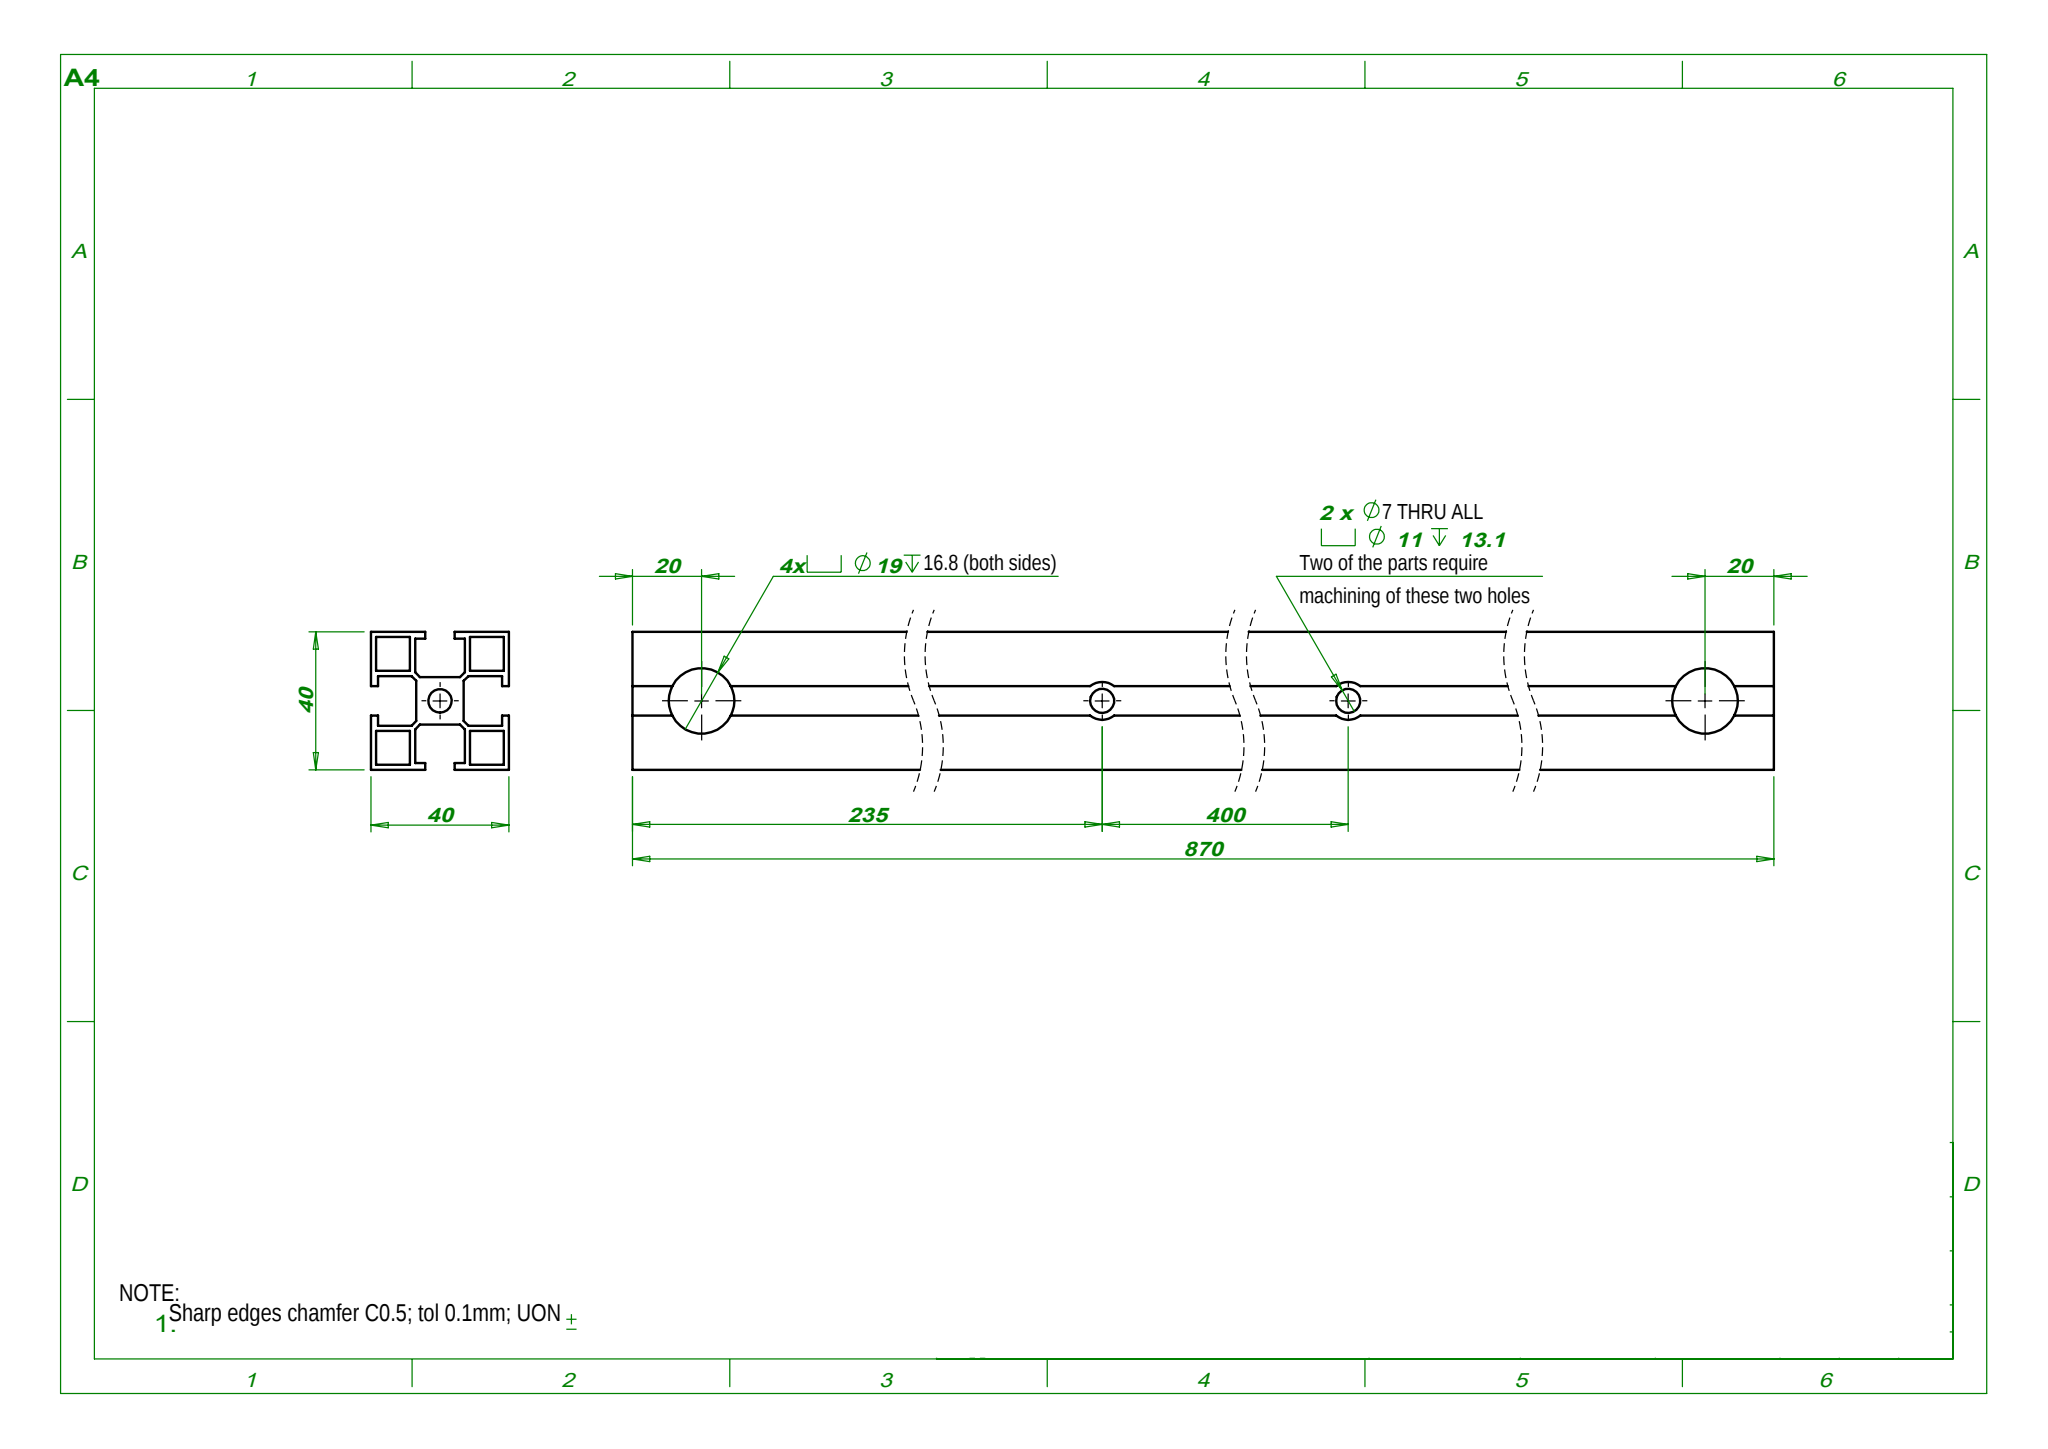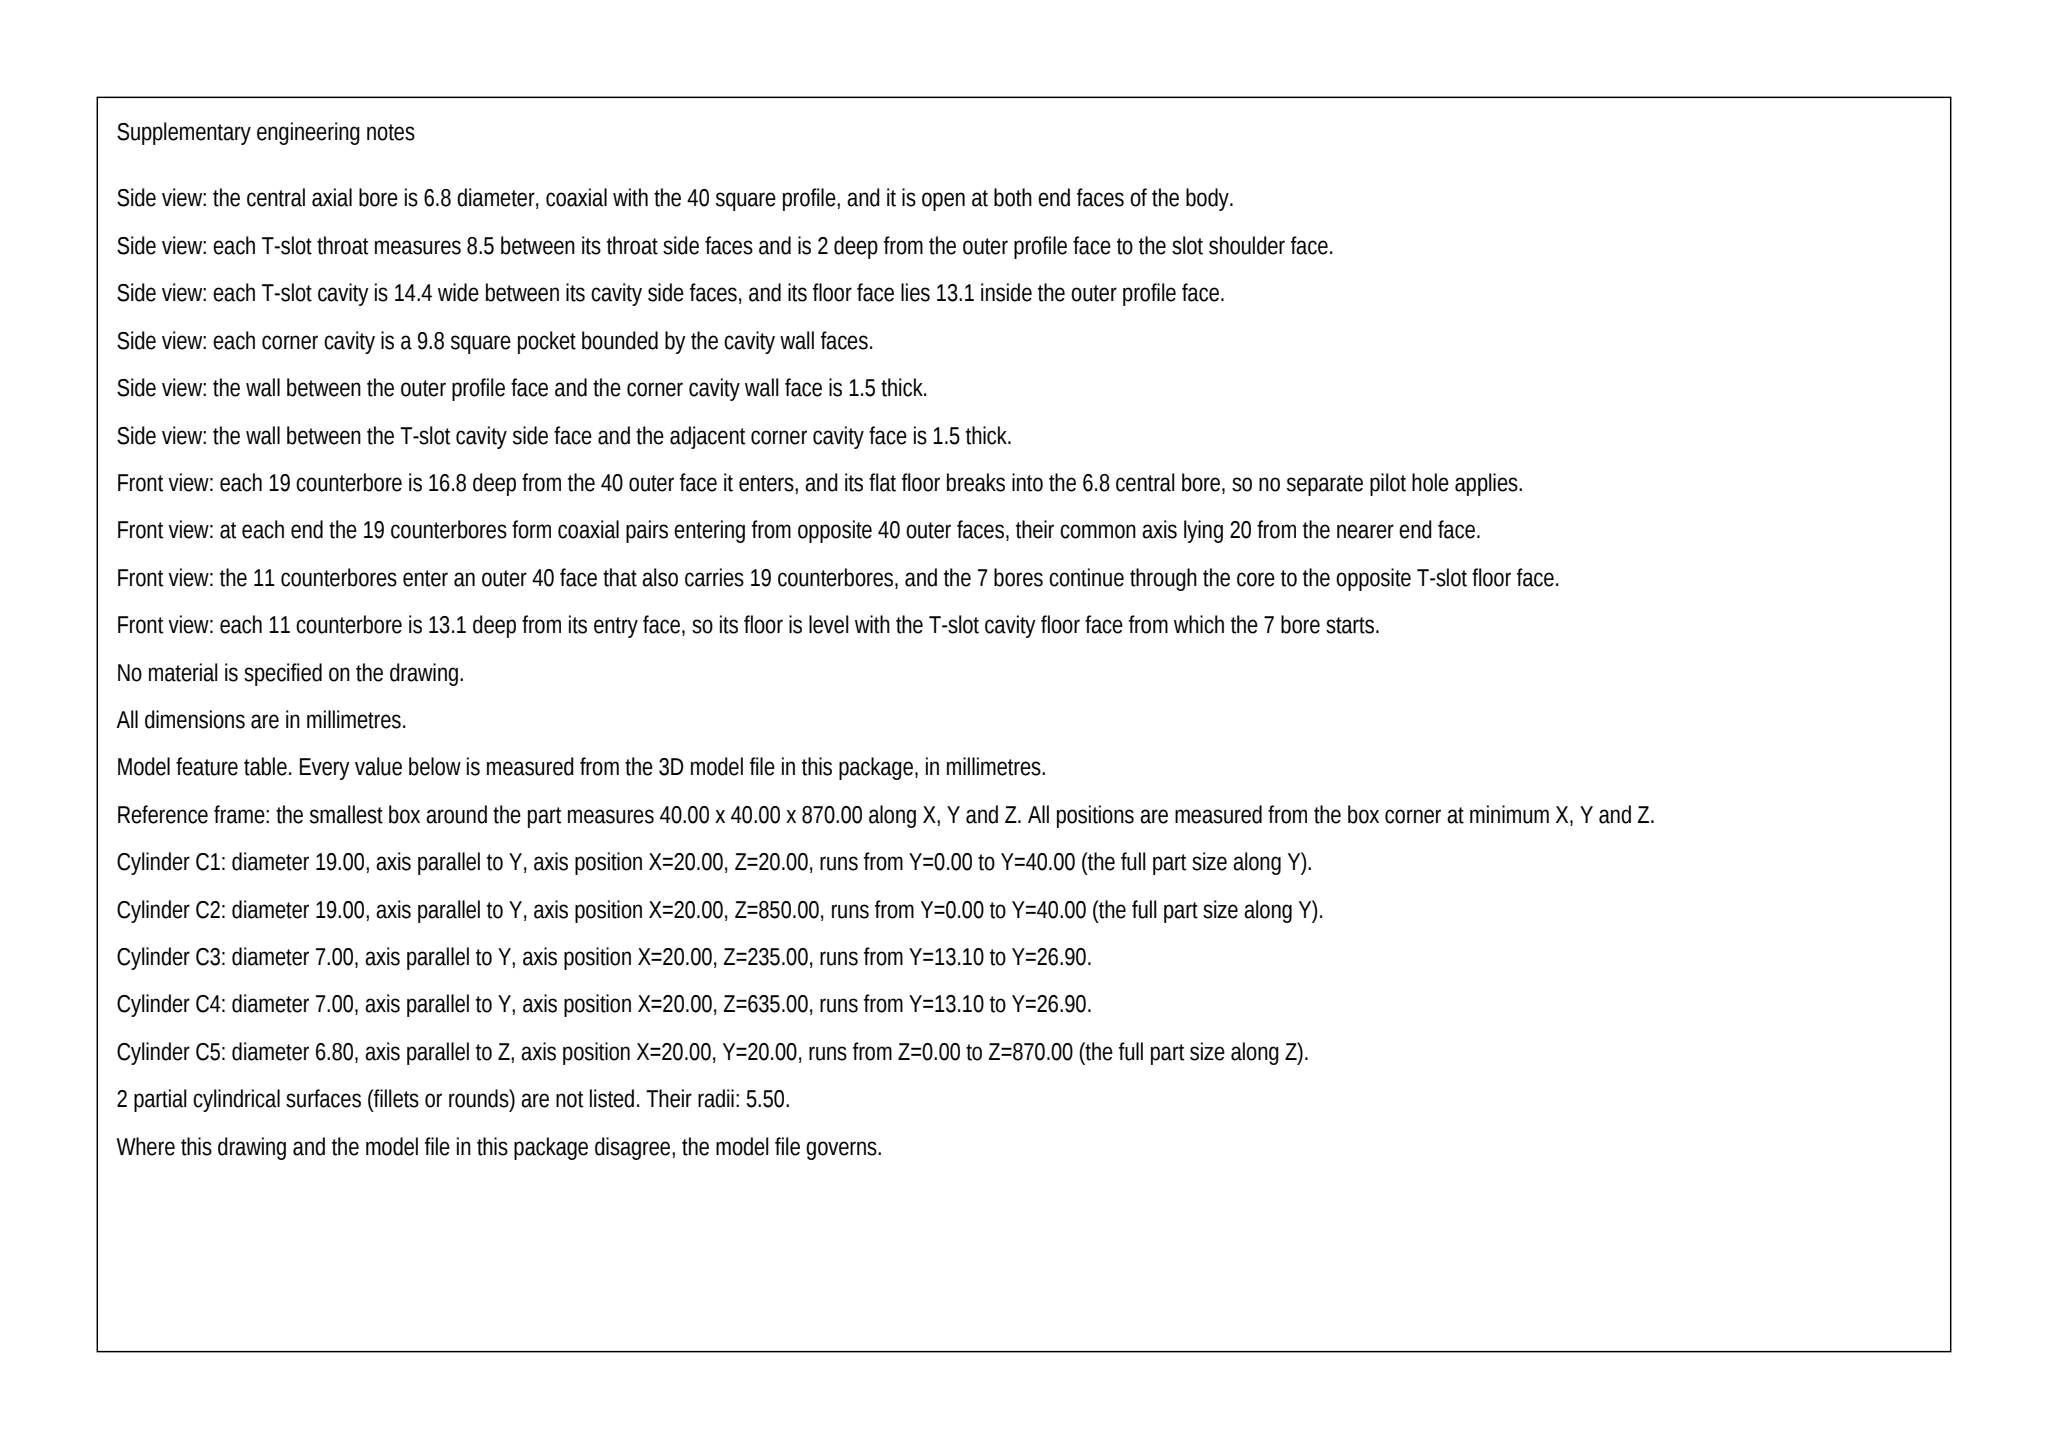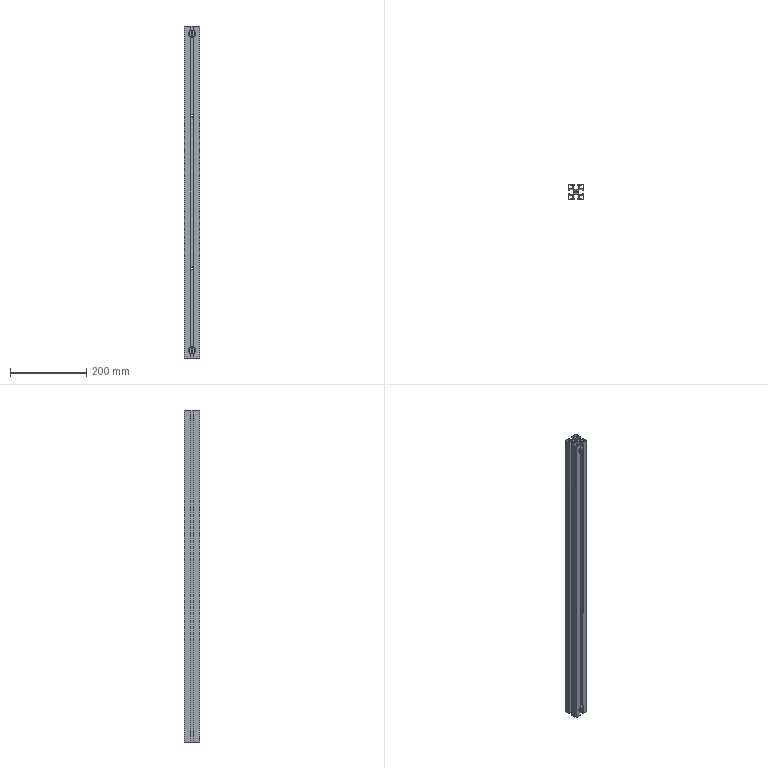Part | SolidWorks | mm | 1 solid | 148 faces | box 40 x 40 x 870 mm | volume 410507 mm3 | plane 126 | cylinder 22 | commonest cylinder face diameters 19 x8 6.8 x6 7 x4 11 x4
Drawing notes:
PROFILE: SLOT OPG 8.5 x 2 LIP, SLOT 14.4 W x 9.3 DP, WALL/RIB 1.5-2 | from the solid: x/y planes 0,1.5,2.0,11.3,12.8,15.75,24.25,27.2,28.7,38.0,38.5,40: opening 24.25-15.75=8.5, lip 2.0, inner slot 27.2-12.8=14.4 wide x 11.3-2.0=9.3 deep, ribs 1.5 thk
Ø6.8 CORE BORE THRU 870, ON C/L 20 x 20 OF SECTION | from the solid: cylinders dia 6.8 axis z at (x=20,y=20), lengths 234.17 x4 + 398.34 x2 spanning full 870 bbox
4x CBORE Ø19 DP 16.8 PILOT HOLE = Ø6.8 CORE BORE THRU | from the solid: Ø19 y-axis cbores at (20,*,20) & (20,*,850) dp 16.8 meet Ø6.8 z core bore at x=20,y=20; no other small dia at ends
2x Ø7 THRU ALL WALLS; C'BORE Ø11 DP 13.1 FROM EA FACE | from the solid: Ø7 cyls axis y at z=235 & 635, segs L=13.8 ea side thru 40 profile; Ø11 c'bore, planes y=13.1 & 26.9 (40-13.1) = depth 13.1 each side
4x SLOT 8.5 WIDE, CTR 20 FROM EDGE, 1 PER FACE | from the solid: x-planes 15.75 & 24.25 (and y-planes 15.75/24.25) give 8.5 opening centered at 20 of 40 bbox
SLOT THROAT WALL 2.0 THK; OUTER WALL & INT RIBS 1.5 THK | from the solid: x/y planes 0-2.0 at slot throat; 0-1.5 and 38.5-40.0 outer wall; ribs 11.3-12.8 and 27.2-28.7 = 1.5
build123d program:
from build123d import *

# Parameters (mm, degrees)
SKETCH1_R                                       = 3.4
SKETCH1_W                                       = 9.8
SKETCH1_H                                       = 9.8
BOSS_EXTRUDE1_DEPTH                             = 435
SKETCH6_R                                       = 9.5
CUT_EXTRUDE1_DEPTH                              = 16.8
MIRROR3_COPY_1_SKETCH_R                         = 9.5
MIRROR3_COPY_1_DEPTH                            = 16.8
M6_HEX_SOCKET_HEAD_CAP_SCREW_CBORE1_D           = 7
M6_HEX_SOCKET_HEAD_CAP_SCREW_CBORE1_CBORE_D     = 11
M6_HEX_SOCKET_HEAD_CAP_SCREW_CBORE1_CBORE_DEPTH = 13.1


with BuildPart() as part:
    # Sketch1 → Boss-Extrude1 (new, symmetric)
    with BuildSketch(Plane.XY):
        Polygon((-4.25, 20), (-20, 20), (-20, 4.25), (-18, 4.25), (-18, 7.2), (-8.261, 7.2), (-6.9, 5.839), (-6.9, -5.839), (-8.261, -7.2), (-18, -7.2), (-18, -4.25), (-20, -4.25), (-20, -20), (-4.25, -20), (-4.25, -18), (-7.2, -18), (-7.2, -8.261), (-5.839, -6.9), (5.839, -6.9), (7.2, -8.261), (7.2, -18), (4.25, -18), (4.25, -20), (20, -20), (20, -4.25), (18, -4.25), (18, -7.2), (8.261, -7.2), (6.9, -5.839), (6.9, 5.839), (8.261, 7.2), (18, 7.2), (18, 4.25), (20, 4.25), (20, 20), (4.25, 20), (4.25, 18), (7.2, 18), (7.2, 8.261), (5.839, 6.9), (-5.839, 6.9), (-7.2, 8.261), (-7.2, 18), (-4.25, 18), align=None)
        with Locations(Location((0, 0, 0), (0, 0, 180))):
            Circle(SKETCH1_R, mode=Mode.SUBTRACT)
        with Locations((-13.6, 13.6)):
            Rectangle(SKETCH1_W, SKETCH1_H, mode=Mode.SUBTRACT)
        with Locations((13.6, 13.6)):
            Rectangle(SKETCH1_W, SKETCH1_H, mode=Mode.SUBTRACT)
        with Locations((13.6, -13.6)):
            Rectangle(SKETCH1_W, SKETCH1_H, mode=Mode.SUBTRACT)
        with Locations((-13.6, -13.6)):
            Rectangle(SKETCH1_W, SKETCH1_H, mode=Mode.SUBTRACT)
    extrude(amount=BOSS_EXTRUDE1_DEPTH, both=True)

    # Sketch6 → Cut-Extrude1 (cut)
    with BuildSketch(Plane(origin=(0, 20, 0), x_dir=(1, 0, 0), z_dir=(0, 1, 0))):
        with Locations(Location((0, -415, 0), (0, 0, 150.406))):
            Circle(SKETCH6_R)
    cut_extrude1 = extrude(amount=-CUT_EXTRUDE1_DEPTH, mode=Mode.SUBTRACT)

    # Mirror2: Cut-Extrude1 across plane
    add(cut_extrude1.mirror(Plane.ZX), mode=Mode.SUBTRACT)

    # Mirror3: Cut-Extrude1 across plane
    add(cut_extrude1.mirror(Plane.XY), mode=Mode.SUBTRACT)

    # Mirror3 copy 1 sketch → Mirror3 copy 1 (cut)
    with BuildSketch(Plane.XZ.offset(20)):
        with Locations(Location((0, -415, 0), (0, 0, 150.406))):
            Circle(MIRROR3_COPY_1_SKETCH_R)
    extrude(amount=-MIRROR3_COPY_1_DEPTH, mode=Mode.SUBTRACT)

    # M6 Hex Socket Head Cap Screw CBORE1 (through all)
    with Locations(Plane(origin=(0, 20, 0), x_dir=(1, 0, 0), z_dir=(0, 1, 0))):
        with Locations((0, 200), (0, -200)):
            CounterBoreHole(M6_HEX_SOCKET_HEAD_CAP_SCREW_CBORE1_D / 2, M6_HEX_SOCKET_HEAD_CAP_SCREW_CBORE1_CBORE_D / 2, M6_HEX_SOCKET_HEAD_CAP_SCREW_CBORE1_CBORE_DEPTH)


solid = part.part